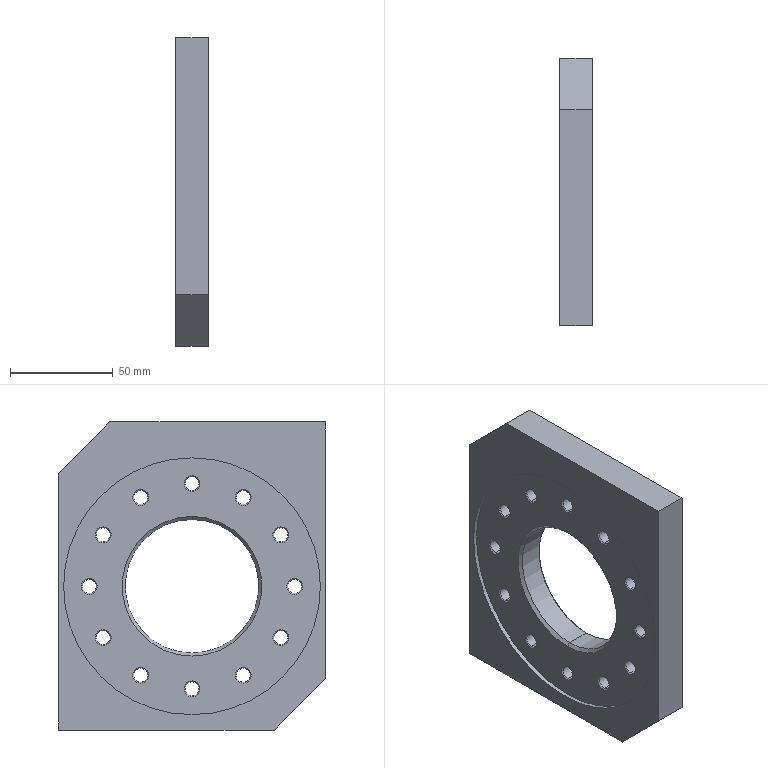Component | SolidWorks | THK-A1022DrivenWheelMountingPlateLeft-1 | 1 solid | 89 faces | box 16 x 130 x 150 mm | volume 224495 mm3 | cone 52 | cylinder 28 | plane 9 | commonest cylinder face diameters 6.8 x24 125 x2 65 x2 | material 45
build123d program:
from build123d import *

# Parameters (mm, degrees)
SKETCH1_W           = 150
SKETCH1_H           = 130
BOSS_EXTRUDE1_DEPTH = 8
SKETCH2_R           = 32.5
CUT_EXTRUDE1_DEPTH  = 101.529
SKETCH3_R           = 62.5
CUT_EXTRUDE2_DEPTH  = 2
M8_TAPPED_HOLE1_D   = 6.8
CHAMFER1_SIZE       = 25
CHAMFER2_SIZE       = 1.5
CHAMFER3_SIZE       = 1
CHAMFER4_SIZE       = 0.5
CHAMFER5_SIZE       = 25


with BuildPart() as part:
    # Sketch1 → Boss-Extrude1 (new, symmetric)
    with BuildSketch(Plane(origin=(0, 0, 0), x_dir=(0, 0, -1), z_dir=(1, 0, 0))):
        Rectangle(SKETCH1_W, SKETCH1_H)
    extrude(amount=BOSS_EXTRUDE1_DEPTH, both=True)

    # Sketch2 → Cut-Extrude1 (cut, through all)
    with BuildSketch(Plane.ZY.offset(8)):
        with Locations((-5, 0)):
            Circle(SKETCH2_R)
    extrude(amount=-CUT_EXTRUDE1_DEPTH, mode=Mode.SUBTRACT)

    # Sketch3 → Cut-Extrude2 (cut)
    with BuildSketch(Plane.ZY.offset(8)):
        with Locations((-5, 0)):
            Circle(SKETCH3_R)
    extrude(amount=-CUT_EXTRUDE2_DEPTH, mode=Mode.SUBTRACT)

    # M8 Tapped Hole1 (through all)
    with Locations(Plane.ZY.offset(6)):
        with Locations((-5, 50), (20, 43.301), (38.301, 25), (45, 0), (38.301, -25), (20, -43.301), (-5, -50), (-30, -43.301), (-48.301, -25), (-55, 0), (-48.301, 25), (-30, 43.301)):
            Hole(M8_TAPPED_HOLE1_D / 2)

    # Chamfer1
    chamfer1_edges = [part.edges().sort_by_distance(p)[0] for p in [
        (0, -65, -75),
    ]]
    chamfer(chamfer1_edges, length=CHAMFER1_SIZE)

    # Chamfer2
    chamfer2_edges = [part.edges().sort_by_distance(p)[0] for p in [
        (-6, 0, -37.5),
    ]]
    chamfer(chamfer2_edges, length=CHAMFER2_SIZE)

    # Chamfer3
    chamfer3_edges = [part.edges().sort_by_distance(p)[0] for p in [
        (8, 0, -37.5),
    ]]
    chamfer(chamfer3_edges, length=CHAMFER3_SIZE)

    # Chamfer4
    chamfer4_edges = [part.edges().sort_by_distance(p)[0] for p in [
        (-6, 43.301, -26.6),
        (8, 43.301, -26.6),
        (-6, 25, -44.901),
        (8, 25, -44.901),
        (-6, 0, -51.6),
        (8, 0, -51.6),
        (-6, -25, -44.901),
        (8, -25, -44.901),
        (-6, -43.301, -26.6),
        (8, -43.301, -26.6),
        (-6, -50, -1.6),
        (8, -50, -1.6),
        (-6, -43.301, 23.4),
        (8, -43.301, 23.4),
        (-6, -25, 41.701),
        (8, -25, 41.701),
        (-6, 0, 48.4),
        (8, 0, 48.4),
        (-6, 25, 41.701),
        (8, 25, 41.701),
        (-6, 43.301, 23.4),
        (8, 43.301, 23.4),
        (-6, 50, -1.6),
        (8, 50, -1.6),
    ]]
    chamfer(chamfer4_edges, length=CHAMFER4_SIZE)

    # Chamfer5
    chamfer5_edges = [part.edges().sort_by_distance(p)[0] for p in [
        (0, 65, 75),
    ]]
    chamfer(chamfer5_edges, length=CHAMFER5_SIZE)


solid = part.part

# Placed as in the assembly
solid = solid.moved(Location((-65, -95, -1324), (0, 0, 0)))